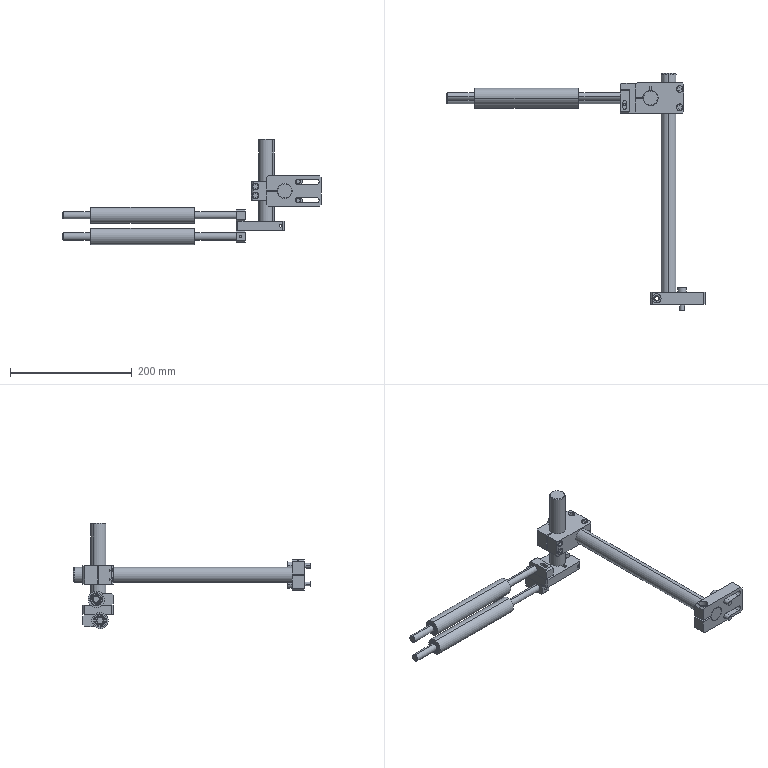Assembly | SolidWorks | mm | 21 component files | 21 solids | 409 faces | box 425 x 390 x 173.5 mm | volume 655029 mm3 | plane 191 | cylinder 182 | cone 36 | commonest cylinder face diameters 12 x24 15 x18 6 x18 21 x16 18 x16 25 x14 11 x10 6.6 x10
Bill of materials:
6801 | 4 |  | Short thick annular ring with a central through bore; the visible end face has a narrow concentric annular groove between the inner and outer rims. It looks like a simplified ring/bearing-style body.
8TC-A15004-90-01A | 1 | A3 | Rectangular block with chamfered corners, a large round through bore, a narrow slit running from the bore to one short edge, and two parallel elongated through slots with rounded ends on the opposite side of the bore. A small cross hole passes through the split portion.
8TC-A15004-90-02A | 1 | Chrome Plated Rod | Plain solid cylindrical rod with flat ends and a long length relative to its diameter.
8TC-A15004-90-03A | 1 | #45 | Rectangular block with two large through bores on perpendicular axes, each with a narrow slit to the outer surface. It has two smaller through holes at one end and small cross holes running through the split regions. The corners are chamfered.
8TC-A15004-90-07A | 1 | Chrome Plated Rod | Plain solid cylindrical pin or rod, shorter and stockier than unnamed part, with flat ends.
8TC-A15004-90-08A | 1 | A6061 | Thick rectangular plate with chamfered corners and a large round through bore, opened to one edge by a wide straight slot. A short round-ended slot extends from the bore on the opposite side. It has two small through holes near the far edge and a small cross hole through the edge face that intersects the open slot.
8TC-A15004-90-09A | 2 | A6061 | Rectangular block with chamfered long edges, a large round through bore through the long side face, an elongated rounded-end slot through the top face, and a small round hole in one end face.
8TC-A15004-90-10A | 2 | Hard Chrome Plated Rod | Long, slender solid cylindrical rod with flat ends. Two faint circumferential lines divide its length into three segments.
8TC-A15004-90-11A | 2 | Brass | Straight, thin-walled cylindrical tube with an open bore running the full length and plain square-cut ends.
M6x20HexSocketCap | 2 | #45 | Cylindrical-headed fastener-like part: a flat-topped cylindrical head with a hexagonal socket recess, on a shorter plain cylindrical shank with a chamfered tip.
M6x30HexSocketCap | 2 | #45 | Cylindrical-headed fastener-like part with a hexagonal socket in the head and a long plain cylindrical shank with a chamfered tip. The shank is proportionally longer than unnamed part's.
M8x30HexSocketCap | 2 | #45 | Headed pin: a cylindrical head on a smaller plain cylindrical shank with a chamfered free end.
Mates:
1. coincident | 8TC-A15004-90-01A-1 face at (0, -10, 0) dir (0, -1, 0) | 8TC-A15004-90-02A-1 face at (-15, -10, 0) dir (0, -1, 0)
2. concentric | 8TC-A15004-90-01A-1 face at (-15, -10, 0) dir (0, 1, 0) r 12.5 | 8TC-A15004-90-02A-1 face at (-15, -10, 0) dir (0, 1, 0) r 12.5
3. concentric | 8TC-A15004-90-02A-1 face at (-15, -10, 0) dir (0, 1, 0) r 12.5 | 8TC-A15004-90-03A-1 face at (-15, 304.3, 0) dir (0, 1, 0) r 12.5
4. parallel | 8TC-A15004-90-01A-1 face at (-45, 10, 25) dir (-1, 0, 0) | 8TC-A15004-90-03A-1 face at (10, 354.3, 15) dir (1, 0, 0)
5. distance | 8TC-A15004-90-03A-1 face at (-30, 354.3, 0) dir (0, 1, 0) | 8TC-A15004-90-02A-1 face at (-15, 370, 0) dir (0, 1, 0)
6. concentric | 8TC-A15004-90-03A-1 face at (-45, 329.3, -15) dir (0, 0, 1) r 12.5 | 8TC-A15004-90-07A-1 face at (-45, 329.3, 85) dir (0, 0, -1) r 12.5
7. coincident | 8TC-A15004-90-03A-1 face at (3, 347.6, 8.6) dir (0, 0, 1) | M6x20HexSocketCap-1 face at (5.39, 348.975, 8.6) dir (0, 0, -1)
8. concentric | 8TC-A15004-90-03A-1 face at (3, 344.3, 15) dir (0, 0, 1) r 3.3 | M6x20HexSocketCap-1 face at (3, 344.3, -11.4) dir (0, 0, -1) r 3
9. coincident | 8TC-A15004-90-03A-1 face at (3, 317.6, 8.6) dir (0, 0, 1) | M6x20HexSocketCap-2 face at (5.39, 318.975, 8.6) dir (0, 0, -1)
10. concentric | 8TC-A15004-90-03A-1 face at (3, 314.3, 15) dir (0, 0, 1) r 3.3 | M6x20HexSocketCap-2 face at (3, 314.3, -11.4) dir (0, 0, -1) r 3
11. concentric | 8TC-A15004-90-03A-1 face at (-63, 304.3, 7.5) dir (0, -1, 0) r 3.3 | M6x30HexSocketCap-1 face at (-63, 340.7, 7.5) dir (0, 1, 0) r 3
12. coincident | 8TC-A15004-90-03A-1 face at (-63, 310.7, 4.2) dir (0, -1, 0) | M6x30HexSocketCap-1 face at (-68.25, 310.7, 7.5) dir (0, 1, 0)
13. coincident | M6x30HexSocketCap-1 face at (-63, 304.7, 7.5) dir (0, -1, 0) | M6x30HexSocketCap-2 face at (-63, 304.7, -7.5) dir (0, -1, 0)
14. concentric | 8TC-A15004-90-03A-1 face at (-63, 304.3, -7.5) dir (0, -1, 0) r 3.3 | M6x30HexSocketCap-2 face at (-63, 340.7, -7.5) dir (0, 1, 0) r 3
15. coincident | 8TC-A15004-90-01A-1 face at (0, 10, 0) dir (0, 1, 0) | M8x30HexSocketCap-1 face at (0, 10, 15) dir (0, -1, 0)
16. concentric | 8TC-A15004-90-01A-1 face at (7, -10, 15) dir (0, 1, 0) r 4.5 | M8x30HexSocketCap-1 face at (7, -20, 15) dir (0, -1, 0) r 4
17. concentric | 8TC-A15004-90-01A-1 face at (7, -10, -15) dir (0, 1, 0) r 4.5 | M8x30HexSocketCap-2 face at (7, -20, -15) dir (0, -1, 0) r 4
18. coincident | 8TC-A15004-90-01A-1 face at (0, 10, 0) dir (0, 1, 0) | M8x30HexSocketCap-2 face at (0, 10, -15) dir (0, -1, 0)
19. distance | 8TC-A15004-90-03A-1 face at (10, 354.3, -15) dir (0, 0, -1) | 8TC-A15004-90-07A-1 face at (-45, 329.3, -65) dir (0, 0, -1)
20. concentric | 8TC-A15004-90-07A-1 face at (-45, 329.3, 85) dir (0, 0, -1) r 12.5 | 8TC-A15004-90-08A-1 face at (-45, 329.3, -65) dir (0, 0, 1) r 12.5
21. coincident | 8TC-A15004-90-07A-1 face at (-45, 329.3, -65) dir (0, 0, -1) | 8TC-A15004-90-08A-1 face at (-15, 304.3, -65) dir (0, 0, -1)
22. coincident | 8TC-A15004-90-03A-1 face at (-30, 354.3, 0) dir (0, 1, 0) | 8TC-A15004-90-08A-1 face at (-55, 354.3, -57.5) dir (0, 1, 0)
23. coincident | 8TC-A15004-90-08A-1 face at (-15, 304.3, -65) dir (0, 0, -1) | 8TC-A15004-90-09A-1 face at (-87.5, 334.3, -65) dir (0, 0, 1)
24. coincident | 8TC-A15004-90-08A-1 face at (-95, 304.3, -65) dir (-1, 0, 0) | 8TC-A15004-90-09A-1 face at (-95, 314.3, -65) dir (-1, 0, 0)
25. coincident | 8TC-A15004-90-08A-1 face at (-95, 304.3, -65) dir (-1, 0, 0) | 8TC-A15004-90-09A-2 face at (-95, 344.3, -50) dir (-1, 0, 0)
26. concentric | 8TC-A15004-90-09A-1 face at (-95, 326.3, -75) dir (1, 0, 0) r 6 | 8TC-A15004-90-10A-1 face at (-80, 326.3, -75) dir (-1, 0, 0) r 6
27. coincident | 8TC-A15004-90-09A-1 face at (-80, 314.3, -65) dir (1, 0, 0) | 8TC-A15004-90-10A-1 face at (-80, 326.3, -75) dir (1, 0, 0)
28. concentric | 8TC-A15004-90-09A-2 face at (-95, 332.3, -40) dir (1, 0, 0) r 6 | 8TC-A15004-90-10A-2 face at (-80, 332.3, -40) dir (-1, 0, 0) r 6
29. coincident | 8TC-A15004-90-09A-2 face at (-80, 344.3, -50) dir (1, 0, 0) | 8TC-A15004-90-10A-2 face at (-80, 332.3, -40) dir (1, 0, 0)
30. coincident | 8TC-A15004-90-08A-1 face at (-55, 354.3, -57.5) dir (0, 1, 0) | 8TC-A15004-90-09A-1 face at (-95, 354.3, -65) dir (0, 1, 0)
31. coincident | 8TC-A15004-90-08A-1 face at (-15, 304.3, -50) dir (0, 0, 1) | 8TC-A15004-90-09A-2 face at (-87.5, 324.3, -50) dir (0, 0, -1)
32. coincident | 8TC-A15004-90-08A-1 face at (-55, 304.3, -57.5) dir (0, -1, 0) | 8TC-A15004-90-09A-2 face at (-95, 304.3, -50) dir (0, -1, 0)
33. concentric | 8TC-A15004-90-10A-1 face at (-80, 326.3, -75) dir (-1, 0, 0) r 6 | 8TC-A15004-90-11A-1 face at (-278.626, 326.3, -75) dir (-1, 0, 0) r 8.5
34. coincident | 8TC-A15004-90-10A-1 face at (-333.85, 320.05, -75) dir (-1, 0, 0) | 8TC-A15004-90-11A-1 face at (-333.85, 328.544, -85.257) dir (-1, 0, 0)
35. concentric | 8TC-A15004-90-10A-2 face at (-80, 332.3, -40) dir (-1, 0, 0) r 6 | 8TC-A15004-90-11A-2 face at (-278.626, 332.3, -40) dir (-1, 0, 0) r 8.5
36. coincident | 8TC-A15004-90-11A-1 face at (-333.85, 328.544, -85.257) dir (-1, 0, 0) | 8TC-A15004-90-11A-2 face at (-333.85, 334.544, -50.257) dir (-1, 0, 0)
37. concentric | 8TC-A15004-90-11A-1 face at (-278.626, 326.3, -75) dir (-1, 0, 0) r 10.5 | 6801-1 face at (-167.35, 326.3, -75) dir (1, 0, 0) r 10.5
38. coincident | 8TC-A15004-90-11A-1 face at (-169.85, 328.116, -83.304) dir (1, 0, 0) | 6801-1 face at (-169.85, 326.3, -64.5) dir (-1, 0, 0)
39. concentric | 8TC-A15004-90-10A-2 face at (-80, 332.3, -40) dir (-1, 0, 0) r 6 | 6801-2 face at (-167.35, 332.3, -40) dir (1, 0, 0) r 6
40. coincident | 8TC-A15004-90-11A-2 face at (-169.85, 334.116, -48.304) dir (1, 0, 0) | 6801-2 face at (-169.85, 332.3, -29.5) dir (-1, 0, 0)
41. concentric | 8TC-A15004-90-11A-2 face at (-278.626, 332.3, -40) dir (-1, 0, 0) r 10.5 | 6801-3 face at (-330.35, 332.3, -40) dir (1, 0, 0) r 10.5
42. coincident | 8TC-A15004-90-11A-2 face at (-327.85, 334.116, -48.304) dir (-1, 0, 0) | 6801-3 face at (-327.85, 332.3, -29.5) dir (1, 0, 0)
43. concentric | 8TC-A15004-90-11A-1 face at (-278.626, 326.3, -75) dir (-1, 0, 0) r 10.5 | 6801-4 face at (-330.35, 326.3, -75) dir (1, 0, 0) r 10.5
44. coincident | 8TC-A15004-90-11A-1 face at (-327.85, 328.116, -83.304) dir (-1, 0, 0) | 6801-4 face at (-327.85, 326.3, -64.5) dir (1, 0, 0)